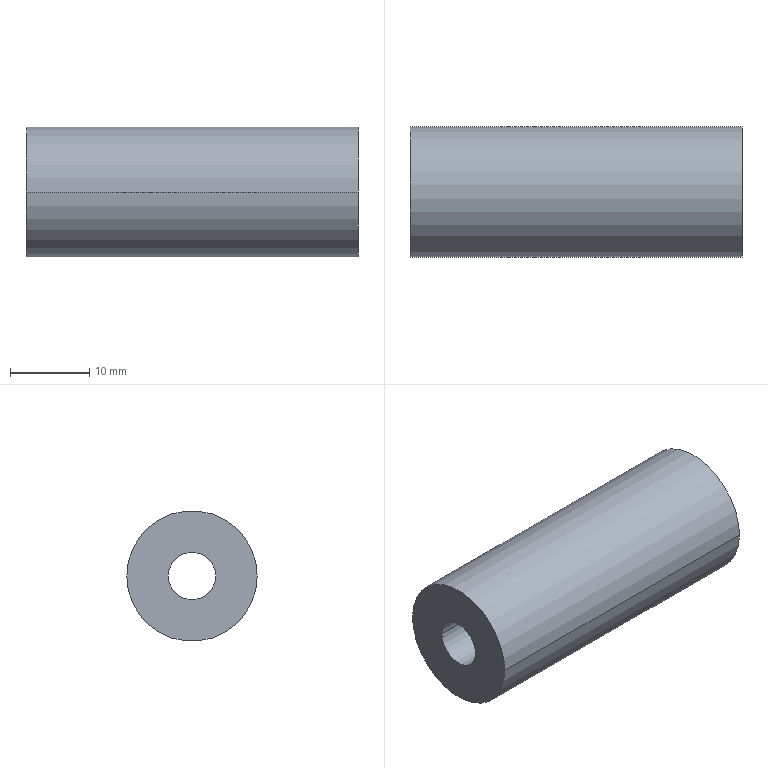Component | SolidWorks | LowerSideBeltXG-XG1-1_6-16-21Coupling-1 | 1 solid | 6 faces | box 42 x 16.5 x 16.5 mm | volume 7793 mm3 | cylinder 4 | plane 2 | commonest cylinder face diameters 6 x2 16.5 x2
build123d program:
from build123d import *

# Parameters (mm, degrees)
SKETCH1_R           = 8.25
SKETCH1_R_2         = 3
BOSS_EXTRUDE1_DEPTH = 21


with BuildPart() as part:
    # Sketch1 → Boss-Extrude1 (new, symmetric)
    with BuildSketch(Plane.XY):
        with Locations(Location((0, 0, 0), (0, 0, 180))):
            Circle(SKETCH1_R)
        with Locations(Location((0, 0, 0), (0, 0, 180))):
            Circle(SKETCH1_R_2, mode=Mode.SUBTRACT)
    extrude(amount=BOSS_EXTRUDE1_DEPTH, both=True)


solid = part.part

# Placed as in the assembly
solid = solid.moved(Location((-145.22, 625, 114), (0, 90, 0)))
STEP:
#1=COLOUR_RGB('',0.7922,0.8196,0.9333);
#2=FILL_AREA_STYLE_COLOUR('',#1);
#3=FILL_AREA_STYLE('',(#2));
#4=SURFACE_STYLE_FILL_AREA(#3);
#5=SURFACE_SIDE_STYLE('',(#4));
#6=SURFACE_STYLE_USAGE(.BOTH.,#5);
#7=PRESENTATION_STYLE_ASSIGNMENT((#6));
#8=CARTESIAN_POINT('',(-4.891,24.488,4.488));
#9=VERTEX_POINT('',#8);
#10=CARTESIAN_POINT('',(-4.891,24.724,4.488));
#11=VERTEX_POINT('',#10);
#12=CARTESIAN_POINT('',(-4.891,24.606,4.488));
#13=DIRECTION('',(1.,0.,-0.));
#14=DIRECTION('',(0.,1.,0.));
#15=AXIS2_PLACEMENT_3D('',#12,#13,#14);
#16=CIRCLE('',#15,0.1181);
#17=EDGE_CURVE('',#9,#11,#16,.T.);
#18=ORIENTED_EDGE('',*,*,#17,.T.);
#19=CARTESIAN_POINT('',(-6.544,24.724,4.488));
#20=VERTEX_POINT('',#19);
#21=CARTESIAN_POINT('',(-4.891,24.724,4.488));
#22=DIRECTION('',(-1.,-0.,0.));
#23=VECTOR('',#22,39.37);
#24=LINE('',#21,#23);
#25=EDGE_CURVE('',#11,#20,#24,.T.);
#26=ORIENTED_EDGE('',*,*,#25,.T.);
#27=CARTESIAN_POINT('',(-6.544,24.488,4.488));
#28=VERTEX_POINT('',#27);
#29=CARTESIAN_POINT('',(-6.544,24.606,4.488));
#30=DIRECTION('',(1.,0.,-0.));
#31=DIRECTION('',(0.,1.,0.));
#32=AXIS2_PLACEMENT_3D('',#29,#30,#31);
#33=CIRCLE('',#32,0.1181);
#34=EDGE_CURVE('',#28,#20,#33,.T.);
#35=ORIENTED_EDGE('',*,*,#34,.F.);
#36=CARTESIAN_POINT('',(-4.891,24.488,4.488));
#37=DIRECTION('',(-1.,-0.,0.));
#38=VECTOR('',#37,39.37);
#39=LINE('',#36,#38);
#40=EDGE_CURVE('',#9,#28,#39,.T.);
#41=ORIENTED_EDGE('',*,*,#40,.F.);
#42=EDGE_LOOP('',(#18,#26,#35,#41));
#43=FACE_OUTER_BOUND('',#42,.T.);
#44=CARTESIAN_POINT('',(-4.891,24.606,4.488));
#45=DIRECTION('',(-1.,-0.,0.));
#46=DIRECTION('',(0.,-1.,0.));
#47=AXIS2_PLACEMENT_3D('',#44,#45,#46);
#48=CYLINDRICAL_SURFACE('',#47,0.1181);
#49=ADVANCED_FACE('',(#43),#48,.F.);
#50=CARTESIAN_POINT('',(-4.891,24.931,4.488));
#51=VERTEX_POINT('',#50);
#52=CARTESIAN_POINT('',(-4.891,24.281,4.488));
#53=VERTEX_POINT('',#52);
#54=CARTESIAN_POINT('',(-4.891,24.606,4.488));
#55=DIRECTION('',(1.,0.,-0.));
#56=DIRECTION('',(0.,1.,0.));
#57=AXIS2_PLACEMENT_3D('',#54,#55,#56);
#58=CIRCLE('',#57,0.3248);
#59=EDGE_CURVE('',#51,#53,#58,.T.);
#60=ORIENTED_EDGE('',*,*,#59,.F.);
#61=CARTESIAN_POINT('',(-6.544,24.931,4.488));
#62=VERTEX_POINT('',#61);
#63=CARTESIAN_POINT('',(-4.891,24.931,4.488));
#64=DIRECTION('',(-1.,-0.,0.));
#65=VECTOR('',#64,39.37);
#66=LINE('',#63,#65);
#67=EDGE_CURVE('',#51,#62,#66,.T.);
#68=ORIENTED_EDGE('',*,*,#67,.T.);
#69=CARTESIAN_POINT('',(-6.544,24.281,4.488));
#70=VERTEX_POINT('',#69);
#71=CARTESIAN_POINT('',(-6.544,24.606,4.488));
#72=DIRECTION('',(1.,0.,-0.));
#73=DIRECTION('',(0.,1.,0.));
#74=AXIS2_PLACEMENT_3D('',#71,#72,#73);
#75=CIRCLE('',#74,0.3248);
#76=EDGE_CURVE('',#62,#70,#75,.T.);
#77=ORIENTED_EDGE('',*,*,#76,.T.);
#78=CARTESIAN_POINT('',(-4.891,24.281,4.488));
#79=DIRECTION('',(-1.,-0.,0.));
#80=VECTOR('',#79,39.37);
#81=LINE('',#78,#80);
#82=EDGE_CURVE('',#53,#70,#81,.T.);
#83=ORIENTED_EDGE('',*,*,#82,.F.);
#84=EDGE_LOOP('',(#60,#68,#77,#83));
#85=FACE_OUTER_BOUND('',#84,.T.);
#86=CARTESIAN_POINT('',(-4.891,24.606,4.488));
#87=DIRECTION('',(-1.,-0.,0.));
#88=DIRECTION('',(0.,-1.,0.));
#89=AXIS2_PLACEMENT_3D('',#86,#87,#88);
#90=CYLINDRICAL_SURFACE('',#89,0.3248);
#91=ADVANCED_FACE('',(#85),#90,.T.);
#92=CARTESIAN_POINT('',(-4.891,24.606,4.488));
#93=DIRECTION('',(1.,0.,-0.));
#94=DIRECTION('',(0.,1.,0.));
#95=AXIS2_PLACEMENT_3D('',#92,#93,#94);
#96=CIRCLE('',#95,0.3248);
#97=EDGE_CURVE('',#53,#51,#96,.T.);
#98=ORIENTED_EDGE('',*,*,#97,.T.);
#99=ORIENTED_EDGE('',*,*,#59,.T.);
#100=EDGE_LOOP('',(#98,#99));
#101=FACE_OUTER_BOUND('',#100,.T.);
#102=ORIENTED_EDGE('',*,*,#17,.F.);
#103=CARTESIAN_POINT('',(-4.891,24.606,4.488));
#104=DIRECTION('',(1.,0.,-0.));
#105=DIRECTION('',(0.,1.,0.));
#106=AXIS2_PLACEMENT_3D('',#103,#104,#105);
#107=CIRCLE('',#106,0.1181);
#108=EDGE_CURVE('',#11,#9,#107,.T.);
#109=ORIENTED_EDGE('',*,*,#108,.F.);
#110=EDGE_LOOP('',(#102,#109));
#111=FACE_BOUND('',#110,.T.);
#112=CARTESIAN_POINT('',(-4.891,24.606,4.488));
#113=DIRECTION('',(1.,0.,-0.));
#114=DIRECTION('',(-0.,1.,0.));
#115=AXIS2_PLACEMENT_3D('',#112,#113,#114);
#116=PLANE('',#115);
#117=ADVANCED_FACE('',(#101,#111),#116,.T.);
#118=CARTESIAN_POINT('',(-6.544,24.606,4.488));
#119=DIRECTION('',(1.,0.,-0.));
#120=DIRECTION('',(0.,1.,0.));
#121=AXIS2_PLACEMENT_3D('',#118,#119,#120);
#122=CIRCLE('',#121,0.3248);
#123=EDGE_CURVE('',#70,#62,#122,.T.);
#124=ORIENTED_EDGE('',*,*,#123,.F.);
#125=ORIENTED_EDGE('',*,*,#76,.F.);
#126=EDGE_LOOP('',(#124,#125));
#127=FACE_OUTER_BOUND('',#126,.T.);
#128=ORIENTED_EDGE('',*,*,#34,.T.);
#129=CARTESIAN_POINT('',(-6.544,24.606,4.488));
#130=DIRECTION('',(1.,0.,-0.));
#131=DIRECTION('',(0.,1.,0.));
#132=AXIS2_PLACEMENT_3D('',#129,#130,#131);
#133=CIRCLE('',#132,0.1181);
#134=EDGE_CURVE('',#20,#28,#133,.T.);
#135=ORIENTED_EDGE('',*,*,#134,.T.);
#136=EDGE_LOOP('',(#128,#135));
#137=FACE_BOUND('',#136,.T.);
#138=CARTESIAN_POINT('',(-6.544,24.606,4.488));
#139=DIRECTION('',(1.,0.,-0.));
#140=DIRECTION('',(-0.,1.,0.));
#141=AXIS2_PLACEMENT_3D('',#138,#139,#140);
#142=PLANE('',#141);
#143=ADVANCED_FACE('',(#127,#137),#142,.F.);
#144=ORIENTED_EDGE('',*,*,#67,.F.);
#145=ORIENTED_EDGE('',*,*,#97,.F.);
#146=ORIENTED_EDGE('',*,*,#82,.T.);
#147=ORIENTED_EDGE('',*,*,#123,.T.);
#148=EDGE_LOOP('',(#144,#145,#146,#147));
#149=FACE_OUTER_BOUND('',#148,.T.);
#150=CARTESIAN_POINT('',(-4.891,24.606,4.488));
#151=DIRECTION('',(-1.,-0.,0.));
#152=DIRECTION('',(0.,-1.,0.));
#153=AXIS2_PLACEMENT_3D('',#150,#151,#152);
#154=CYLINDRICAL_SURFACE('',#153,0.3248);
#155=ADVANCED_FACE('',(#149),#154,.T.);
#156=ORIENTED_EDGE('',*,*,#25,.F.);
#157=ORIENTED_EDGE('',*,*,#108,.T.);
#158=ORIENTED_EDGE('',*,*,#40,.T.);
#159=ORIENTED_EDGE('',*,*,#134,.F.);
#160=EDGE_LOOP('',(#156,#157,#158,#159));
#161=FACE_OUTER_BOUND('',#160,.T.);
#162=CARTESIAN_POINT('',(-4.891,24.606,4.488));
#163=DIRECTION('',(-1.,-0.,0.));
#164=DIRECTION('',(0.,-1.,0.));
#165=AXIS2_PLACEMENT_3D('',#162,#163,#164);
#166=CYLINDRICAL_SURFACE('',#165,0.1181);
#167=ADVANCED_FACE('',(#161),#166,.F.);
#168=CLOSED_SHELL('',(#49,#91,#117,#143,#155,#167));
#169=MANIFOLD_SOLID_BREP('',#168);
#170=STYLED_ITEM('',(#7),#169);
#171=(LENGTH_UNIT()NAMED_UNIT(*)SI_UNIT($,.METRE.));
#172=LENGTH_MEASURE_WITH_UNIT(LENGTH_MEASURE(0.0254),#171);
#173=DIMENSIONAL_EXPONENTS(1.,0.,0.,0.,0.,0.,0.);
#174=(CONVERSION_BASED_UNIT('',#172)LENGTH_UNIT()NAMED_UNIT(#173));
#175=UNCERTAINTY_MEASURE_WITH_UNIT(LENGTH_MEASURE(0.00001),#174,'','');
#176=(NAMED_UNIT(*)PLANE_ANGLE_UNIT()SI_UNIT($,.RADIAN.));
#177=(NAMED_UNIT(*)SI_UNIT($,.STERADIAN.)SOLID_ANGLE_UNIT());
#178=(GEOMETRIC_REPRESENTATION_CONTEXT(3)GLOBAL_UNCERTAINTY_ASSIGNED_CONTEXT((#175))GLOBAL_UNIT_ASSIGNED_CONTEXT((#174,#176,#177))REPRESENTATION_CONTEXT('',''));
#179=MECHANICAL_DESIGN_GEOMETRIC_PRESENTATION_REPRESENTATION('',(#170),#178);
#180=PRESENTATION_LAYER_ASSIGNMENT('','',(#170));
#181=CARTESIAN_POINT('',(0.,0.,0.));
#182=DIRECTION('',(0.,0.,1.));
#183=DIRECTION('',(1.,0.,0.));
#184=AXIS2_PLACEMENT_3D('',#181,#182,#183);
#185=(LENGTH_UNIT()NAMED_UNIT(*)SI_UNIT($,.METRE.));
#186=LENGTH_MEASURE_WITH_UNIT(LENGTH_MEASURE(0.0254),#185);
#187=DIMENSIONAL_EXPONENTS(1.,0.,0.,0.,0.,0.,0.);
#188=(CONVERSION_BASED_UNIT('',#186)LENGTH_UNIT()NAMED_UNIT(#187));
#189=UNCERTAINTY_MEASURE_WITH_UNIT(LENGTH_MEASURE(0.00001),#188,'','');
#190=(NAMED_UNIT(*)PLANE_ANGLE_UNIT()SI_UNIT($,.RADIAN.));
#191=(NAMED_UNIT(*)SI_UNIT($,.STERADIAN.)SOLID_ANGLE_UNIT());
#192=(GEOMETRIC_REPRESENTATION_CONTEXT(3)GLOBAL_UNCERTAINTY_ASSIGNED_CONTEXT((#189))GLOBAL_UNIT_ASSIGNED_CONTEXT((#188,#190,#191))REPRESENTATION_CONTEXT('',''));
#193=ADVANCED_BREP_SHAPE_REPRESENTATION('',(#169,#184),#192);